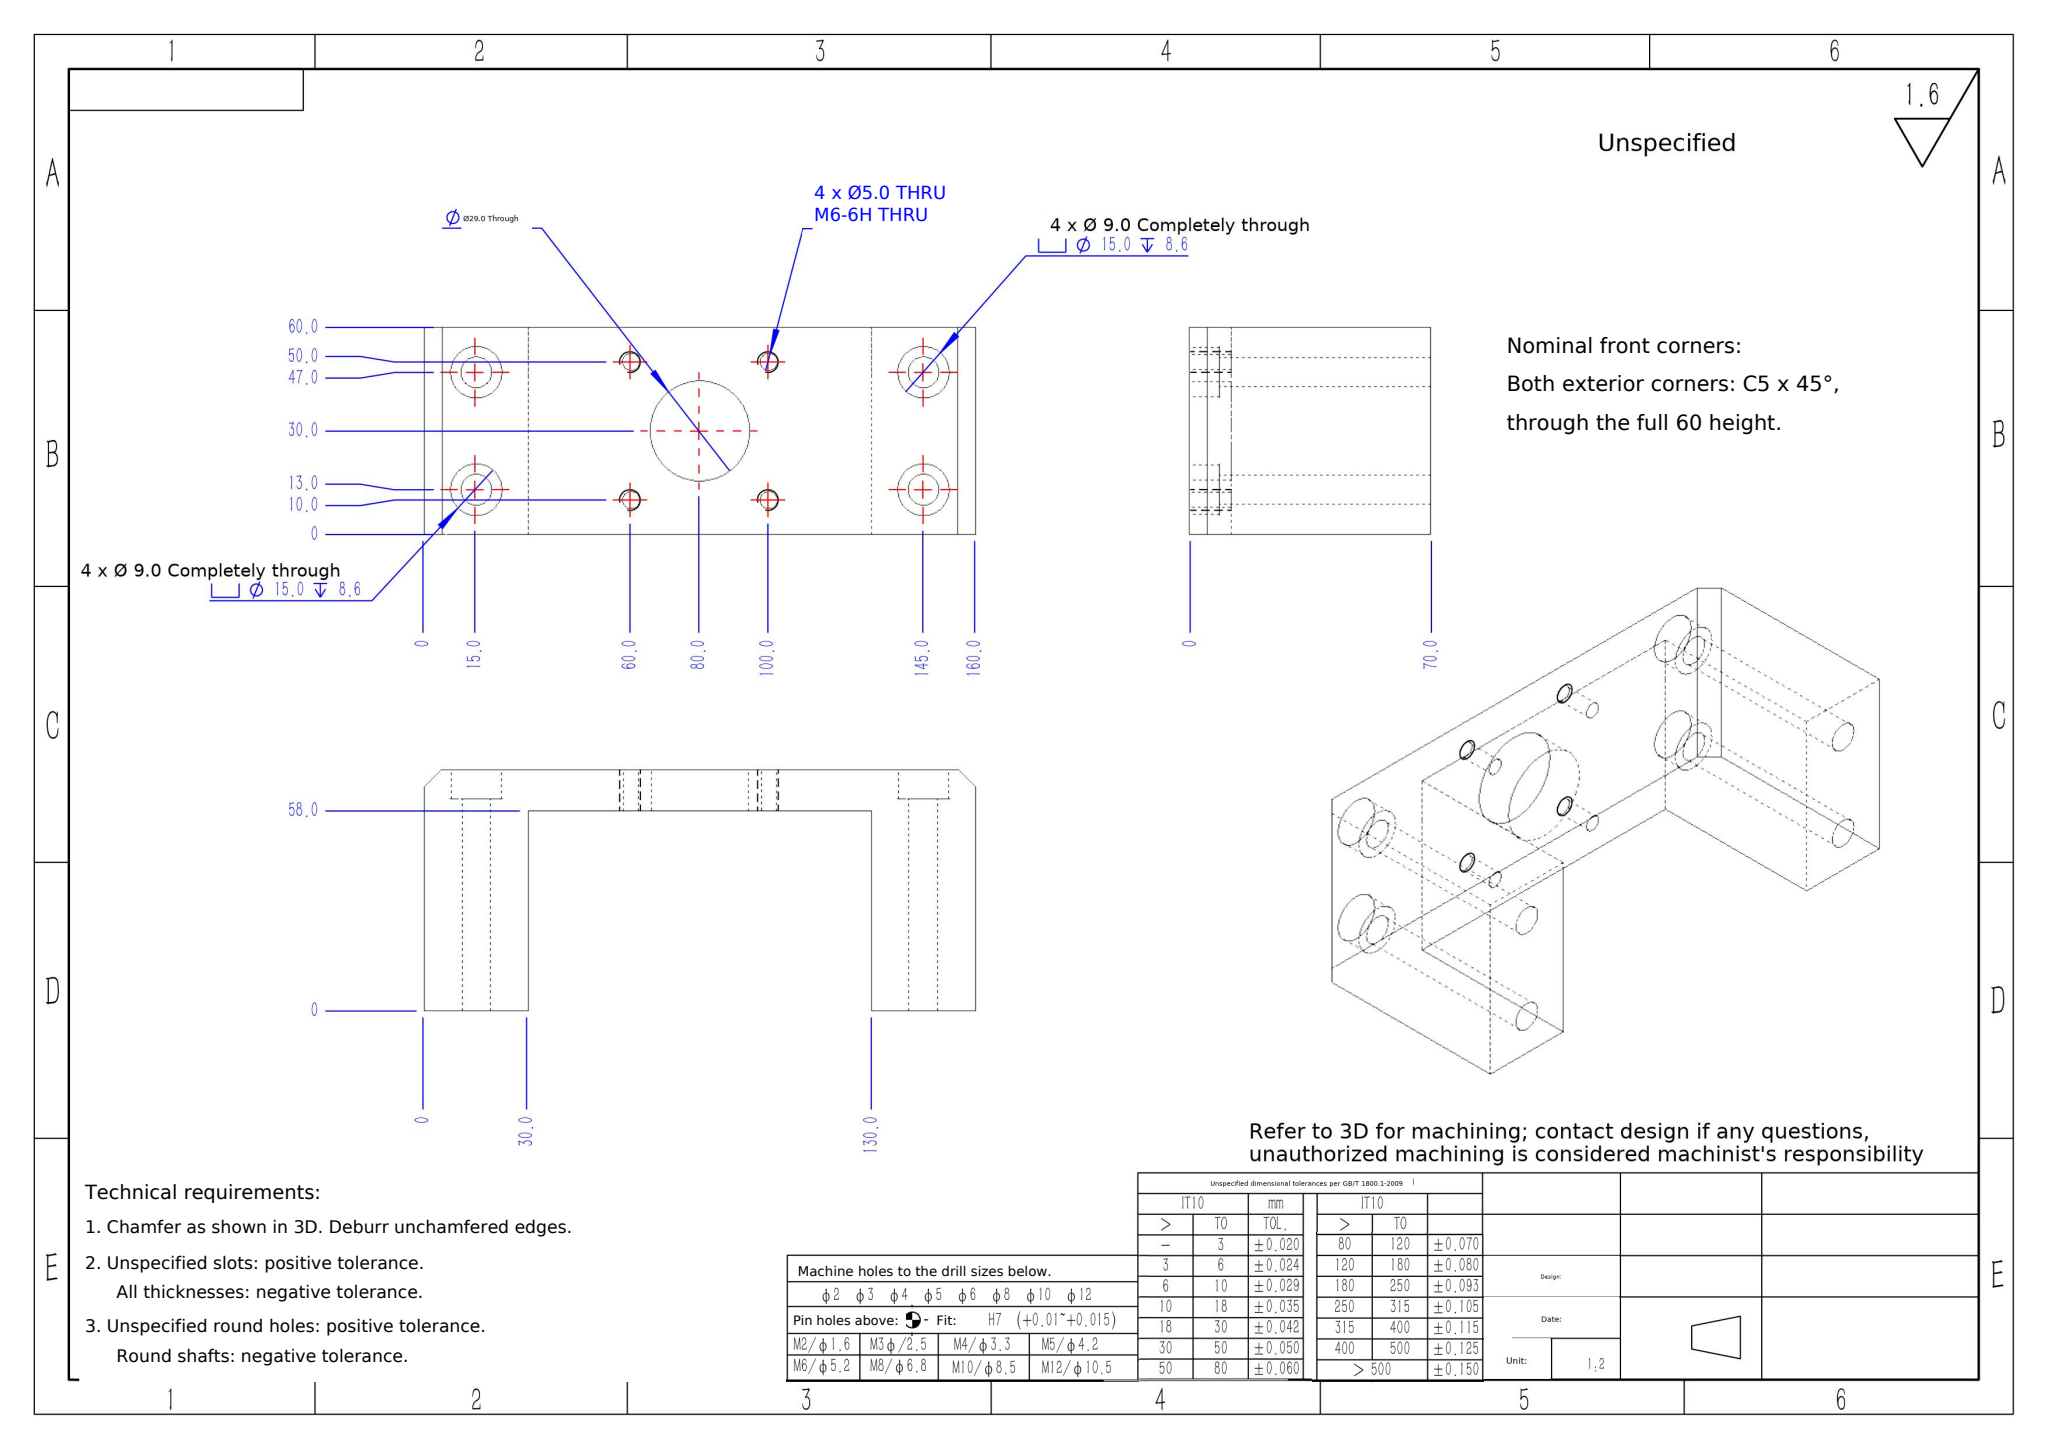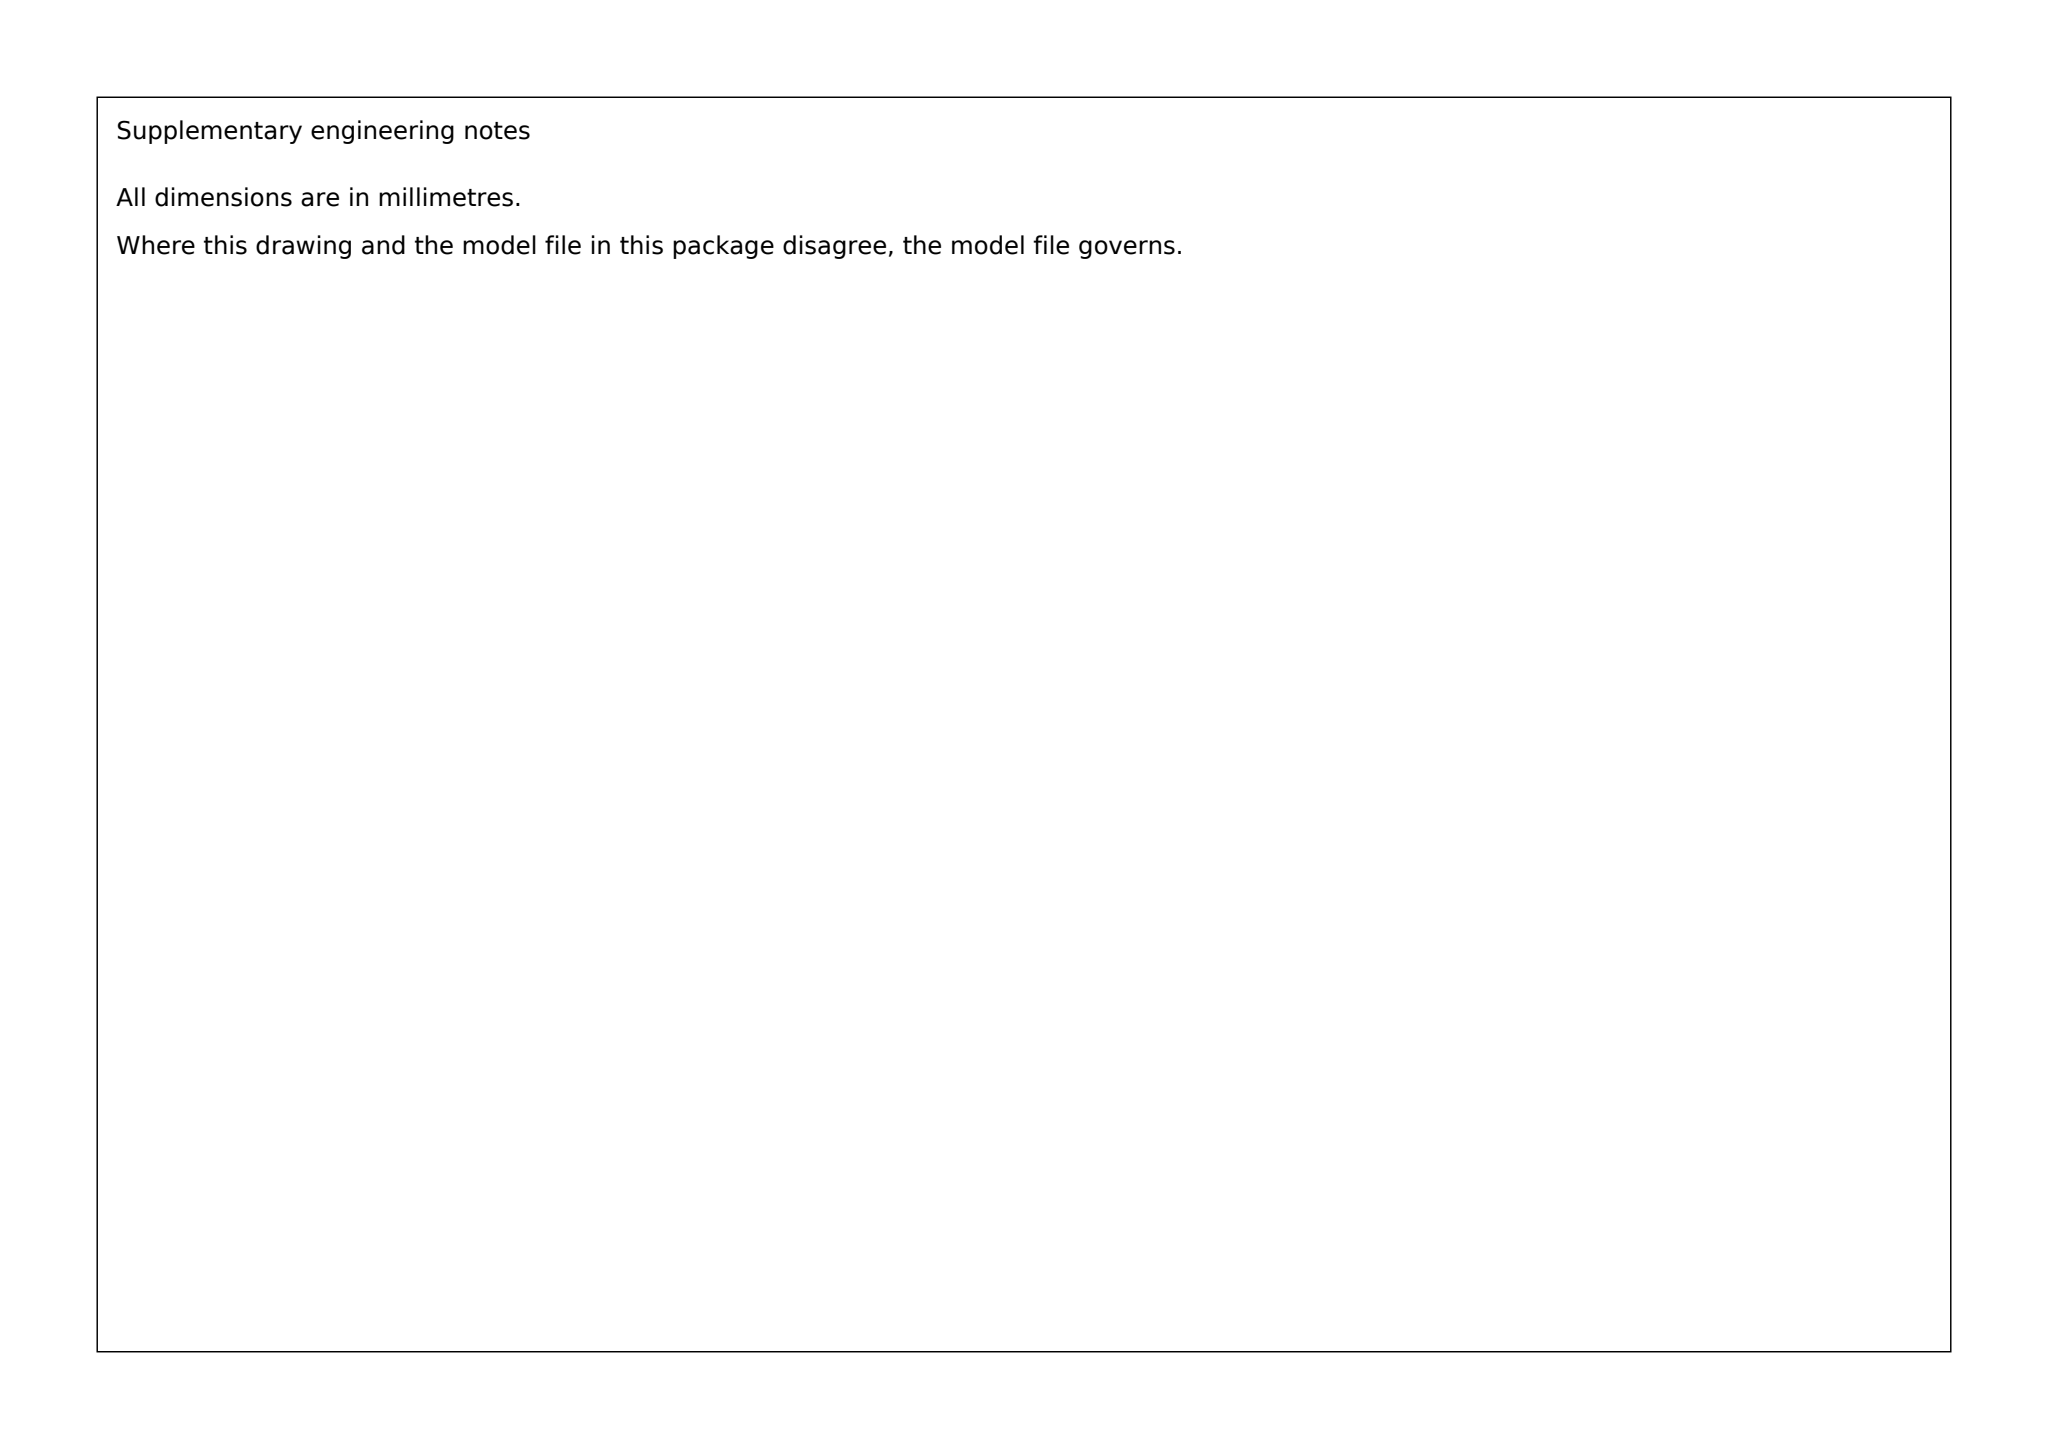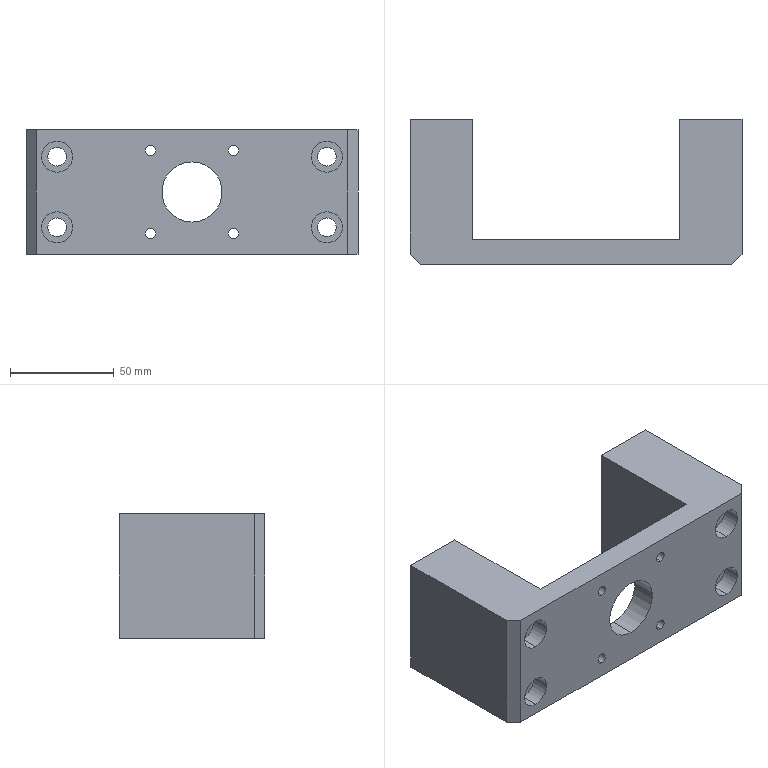Part | SolidWorks | mm | 1 solid | 42 faces | box 160 x 70 x 60 mm | volume 291928 mm3 | cylinder 26 | plane 16 | commonest cylinder face diameters 15 x8 9 x8 5 x8 29 x2
build123d program:
from build123d import *

# Parameters (mm, degrees)
SKETCH1_W                                       = 160
SKETCH1_H                                       = 70
BOSS_EXTRUDE1_DEPTH                             = 30
SKETCH2_W                                       = 100
SKETCH2_H                                       = 58
CUT_EXTRUDE1_DEPTH                              = 113
CHAMFER1_SIZE                                   = 5
SKETCH3_R                                       = 14.5
CUT_EXTRUDE2_DEPTH                              = 113
M6_TAPPED_HOLE1_D                               = 5
M8_HEX_SOCKET_HEAD_CAP_SCREW_CBORE1_D           = 9
M8_HEX_SOCKET_HEAD_CAP_SCREW_CBORE1_CBORE_D     = 15
M8_HEX_SOCKET_HEAD_CAP_SCREW_CBORE1_CBORE_DEPTH = 8.6
MIRROR2_COPY_1_D                                = 9
MIRROR2_COPY_1_CBORE_D                          = 15
MIRROR2_COPY_1_CBORE_DEPTH                      = 8.6


with BuildPart() as part:
    # Sketch1 → Boss-Extrude1 (new, symmetric)
    with BuildSketch(Plane.XY):
        Rectangle(SKETCH1_W, SKETCH1_H)
    extrude(amount=BOSS_EXTRUDE1_DEPTH, both=True)

    # Sketch2 → Cut-Extrude1 (cut)
    with BuildSketch(Plane(origin=(0, 0, -30), x_dir=(-1, 0, 0), z_dir=(0, 0, -1))):
        with Locations((0, 6)):
            Rectangle(SKETCH2_W, SKETCH2_H)
    extrude(amount=-CUT_EXTRUDE1_DEPTH, mode=Mode.SUBTRACT)

    # Chamfer1
    chamfer1_edges = [part.edges().sort_by_distance(p)[0] for p in [
        (80, -35, 0),
        (-80, -35, 0),
    ]]
    chamfer(chamfer1_edges, length=CHAMFER1_SIZE)

    # Sketch3 → Cut-Extrude2 (cut)
    with BuildSketch(Plane.XZ.offset(35)):
        with Locations(Location((0, 0, 0), (0, 0, 270))):
            Circle(SKETCH3_R)
    extrude(amount=-CUT_EXTRUDE2_DEPTH, mode=Mode.SUBTRACT)

    # M6 Tapped Hole1 (through all)
    with Locations(Plane(origin=(0, -35, 0), x_dir=(-1, 0, 0), z_dir=(0, -1, 0))):
        with Locations((20, -20), (20, 20), (-20, 20), (-20, -20)):
            Hole(M6_TAPPED_HOLE1_D / 2)

    # M8 Hex Socket Head Cap Screw CBORE1 (through all)
    with Locations(Plane(origin=(0, -35, 0), x_dir=(-1, 0, 0), z_dir=(0, -1, 0))):
        with Locations((-65, -17)):
            m8_hex_socket_head_cap_screw_cbore1 = CounterBoreHole(M8_HEX_SOCKET_HEAD_CAP_SCREW_CBORE1_D / 2, M8_HEX_SOCKET_HEAD_CAP_SCREW_CBORE1_CBORE_D / 2, M8_HEX_SOCKET_HEAD_CAP_SCREW_CBORE1_CBORE_DEPTH)

    # Mirror1: M8 Hex Socket Head Cap Screw CBORE1 across plane
    add(m8_hex_socket_head_cap_screw_cbore1.mirror(Plane.XY), mode=Mode.SUBTRACT)

    # Mirror2: M8 Hex Socket Head Cap Screw CBORE1 across plane
    add(m8_hex_socket_head_cap_screw_cbore1.mirror(Plane(origin=(0, 0, 0), x_dir=(0, 0, 1), z_dir=(1, 0, 0))), mode=Mode.SUBTRACT)

    # Mirror2 copy 1 (through all)
    with Locations(Plane.XZ.offset(35)):
        with Locations((-65, -17)):
            CounterBoreHole(MIRROR2_COPY_1_D / 2, MIRROR2_COPY_1_CBORE_D / 2, MIRROR2_COPY_1_CBORE_DEPTH)


solid = part.part